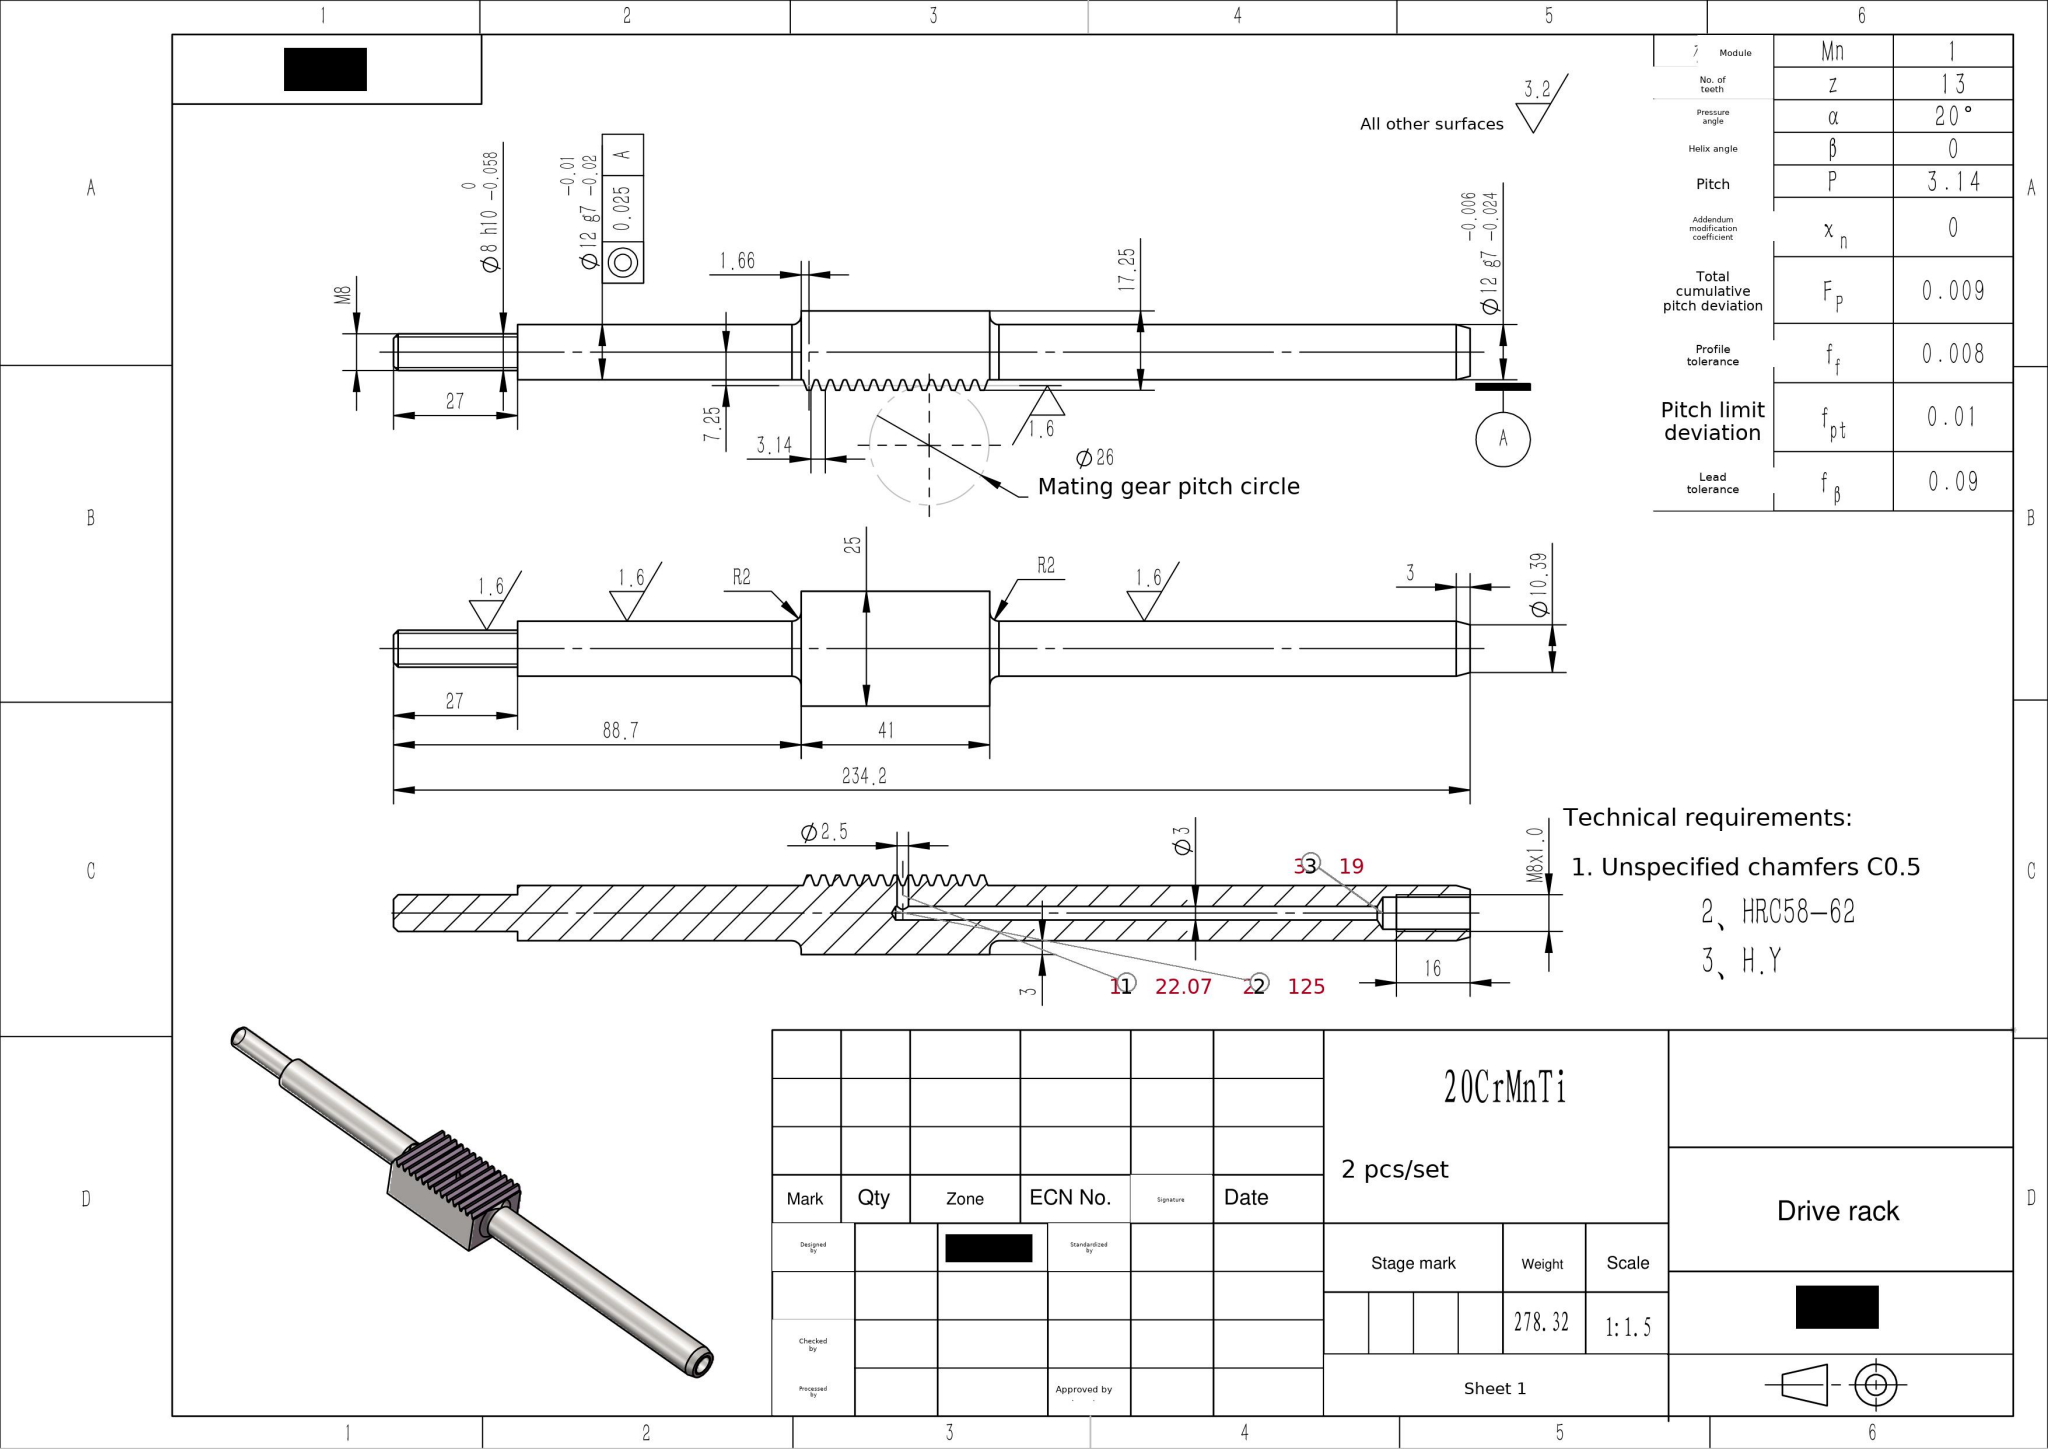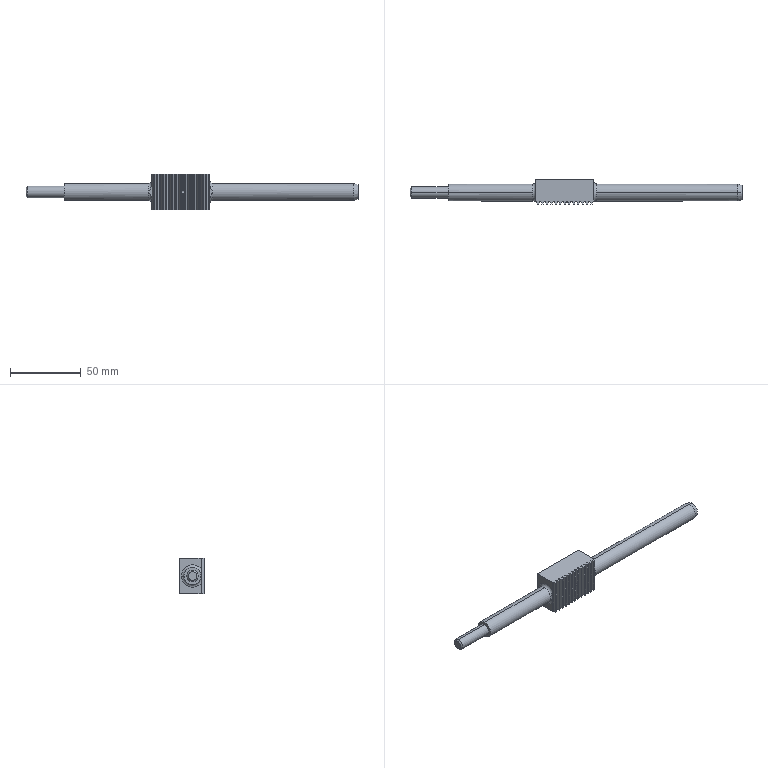Part | SolidWorks | mm | material 20CrMnTi | 1 solid | 116 faces | box 234.2 x 17.25 x 25 mm | volume 35231 mm3 | plane 64 | cylinder 40 | cone 8 | torus 4 | commonest cylinder face diameters 0.6 x28 12 x4 8 x2 7 x2 2.5 x2 3 x2